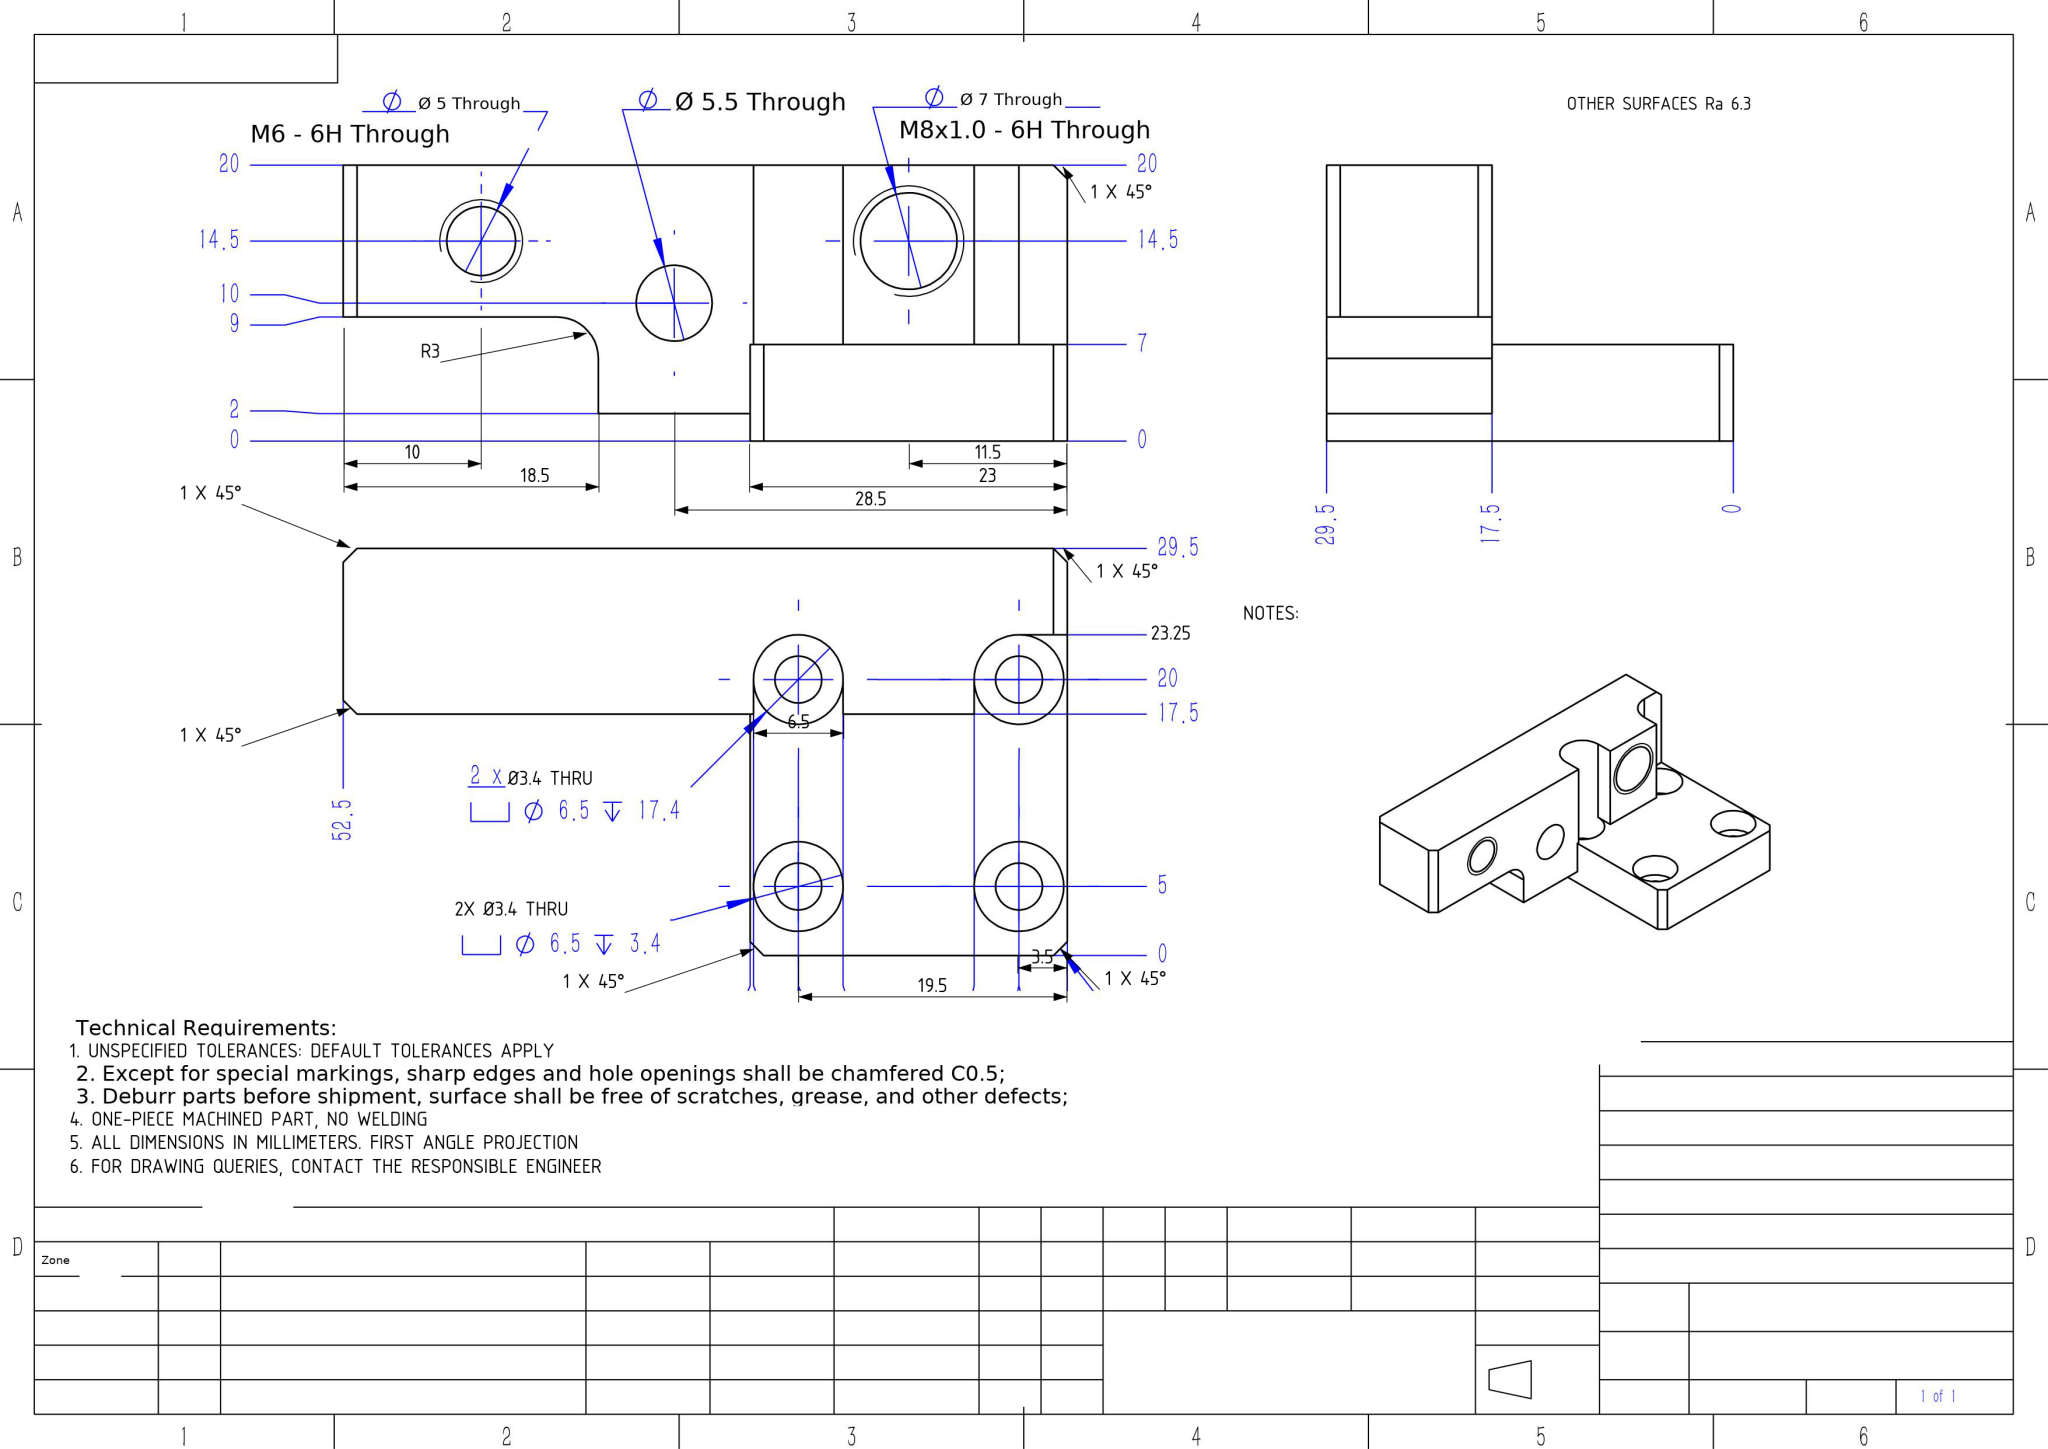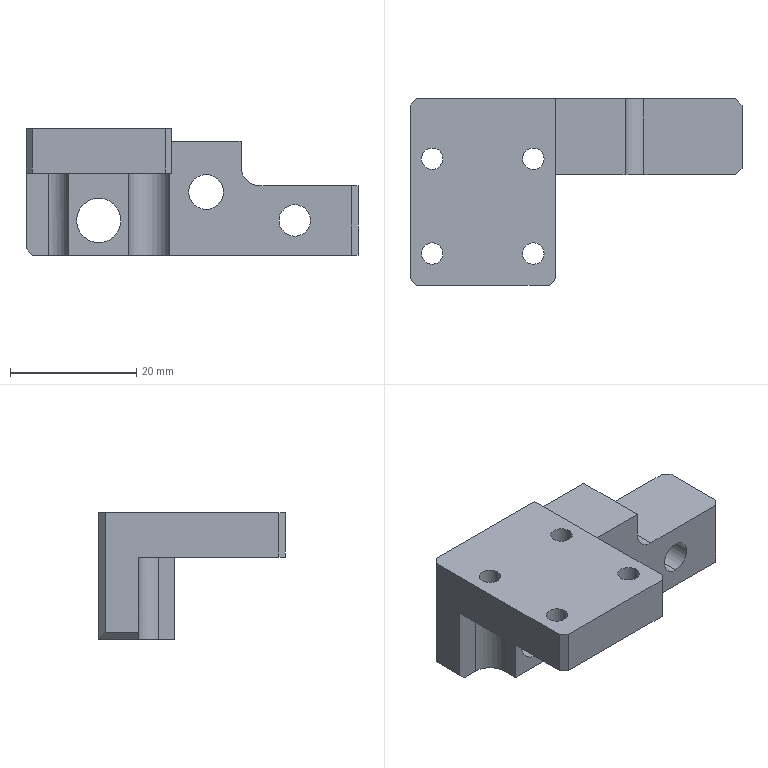Part | NX | mm | 1 solid | 50 faces | box 52.5 x 29.5 x 20 mm | volume 10633 mm3 | plane 27 | cylinder 23 | commonest cylinder face diameters 3.4 x8 6.5 x8 5.5 x2 7 x2 5 x2 6 x1